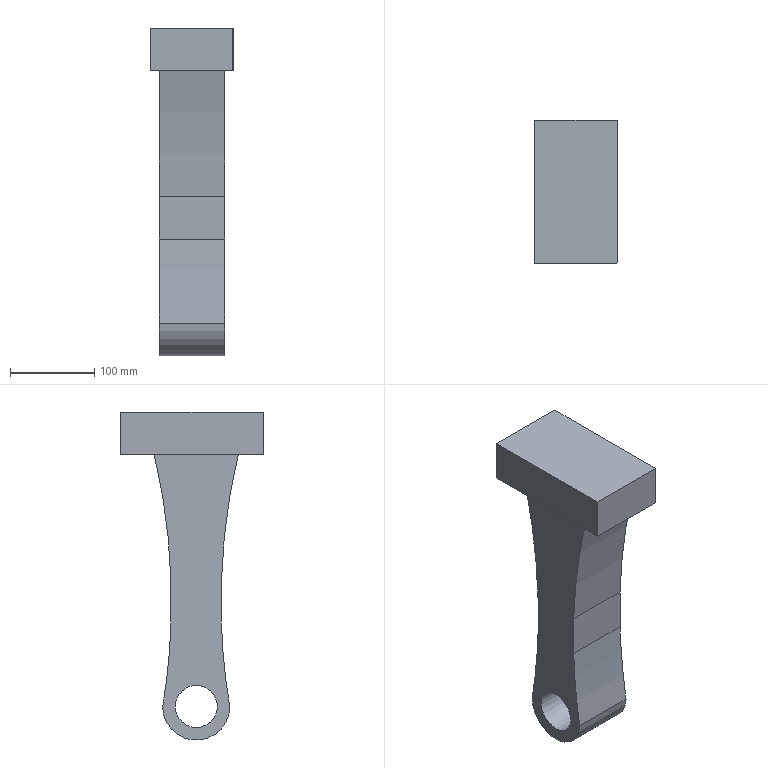Component | NX | UPPER_HAMMER | 1 solid | 18 faces | volume 2512771 mm3 | plane 12 | cylinder 6 | commonest cylinder face diameters 1526.456 x4 80 x1 50 x1